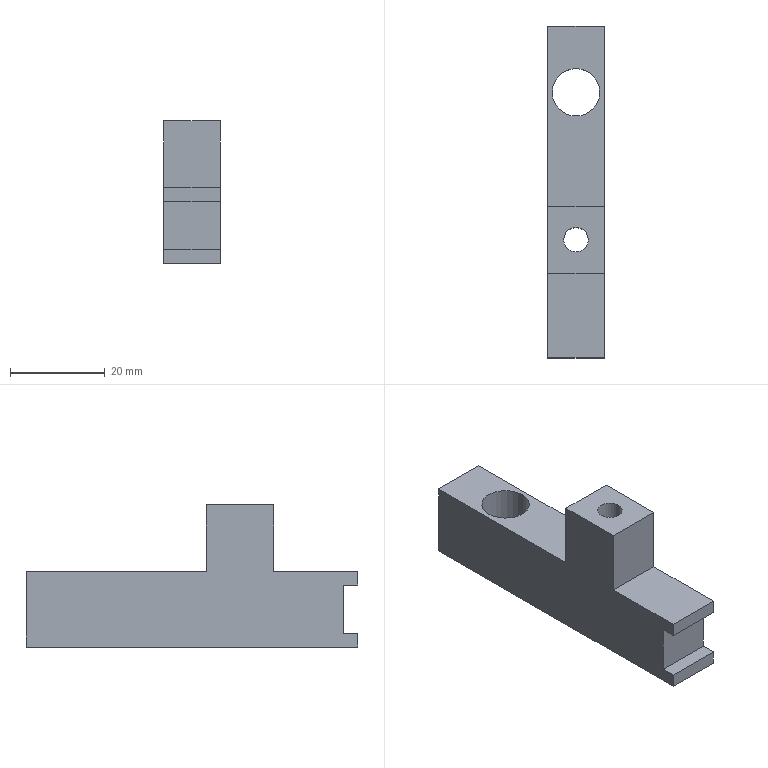Component | SolidWorks | JCT-03-03SwingBlock-1 | 1 solid | 18 faces | box 12 x 70 x 30 mm | volume 13565 mm3 | plane 14 | cylinder 4 | commonest cylinder face diameters 10 x2 5.2 x2
build123d program:
from build123d import *

# Parameters (mm, degrees)
EXTRUDE1_DEPTH     = 6
SKETCH2_R          = 2.6
EXTRUDE2_DEPTH     = 77.394
M10_TAPPED_HOLE1_D = 10


with BuildPart() as part:
    # Sketch1 → Extrude1 (new, symmetric)
    with BuildSketch(Plane(origin=(0, 0, 0), x_dir=(0, 0, -1), z_dir=(1, 0, 0))):
        Polygon((0, 0), (0, 70), (-16, 70), (-16, 32), (-30, 32), (-30, 17.8), (-16, 17.8), (-16, 0), (-13.1, 0), (-13.1, 3), (-2.9, 3), (-2.9, 0), align=None)
    extrude(amount=EXTRUDE1_DEPTH, both=True)

    # Sketch2 → Extrude2 (cut, through all)
    with BuildSketch(Plane.XY.offset(30)):
        with Locations((0, 24.9)):
            Circle(SKETCH2_R)
    extrude(amount=-EXTRUDE2_DEPTH, mode=Mode.SUBTRACT)

    # M10 Tapped Hole1 (through all)
    with Locations(Plane(origin=(0, 0, 0), x_dir=(-1, 0, 0), z_dir=(0, 0, -1))):
        with Locations((0, 56)):
            Hole(M10_TAPPED_HOLE1_D / 2)


solid = part.part

# Placed as in the assembly
solid = solid.moved(Location((7.266, 13.399, 26), (0, 0, 0)))
STEP:
#1=COLOUR_RGB('',0.7922,0.8196,0.9333);
#2=FILL_AREA_STYLE_COLOUR('',#1);
#3=FILL_AREA_STYLE('',(#2));
#4=SURFACE_STYLE_FILL_AREA(#3);
#5=SURFACE_SIDE_STYLE('',(#4));
#6=SURFACE_STYLE_USAGE(.BOTH.,#5);
#7=PRESENTATION_STYLE_ASSIGNMENT((#6));
#8=CARTESIAN_POINT('',(0.4829,2.732,1.654));
#9=VERTEX_POINT('',#8);
#10=CARTESIAN_POINT('',(0.08922,2.732,1.654));
#11=VERTEX_POINT('',#10);
#12=CARTESIAN_POINT('',(0.2861,2.732,1.654));
#13=DIRECTION('',(0.,0.,-1.));
#14=DIRECTION('',(-1.,0.,0.));
#15=AXIS2_PLACEMENT_3D('',#12,#13,#14);
#16=CIRCLE('',#15,0.1969);
#17=EDGE_CURVE('',#9,#11,#16,.T.);
#18=ORIENTED_EDGE('',*,*,#17,.F.);
#19=CARTESIAN_POINT('',(0.4829,2.732,1.024));
#20=VERTEX_POINT('',#19);
#21=CARTESIAN_POINT('',(0.4829,2.732,1.024));
#22=DIRECTION('',(0.,0.,-1.));
#23=VECTOR('',#22,39.37);
#24=LINE('',#21,#23);
#25=EDGE_CURVE('',#9,#20,#24,.T.);
#26=ORIENTED_EDGE('',*,*,#25,.T.);
#27=CARTESIAN_POINT('',(0.08922,2.732,1.024));
#28=VERTEX_POINT('',#27);
#29=CARTESIAN_POINT('',(0.2861,2.732,1.024));
#30=DIRECTION('',(0.,0.,-1.));
#31=DIRECTION('',(-1.,0.,0.));
#32=AXIS2_PLACEMENT_3D('',#29,#30,#31);
#33=CIRCLE('',#32,0.1969);
#34=EDGE_CURVE('',#20,#28,#33,.T.);
#35=ORIENTED_EDGE('',*,*,#34,.T.);
#36=CARTESIAN_POINT('',(0.08922,2.732,1.024));
#37=DIRECTION('',(0.,0.,-1.));
#38=VECTOR('',#37,39.37);
#39=LINE('',#36,#38);
#40=EDGE_CURVE('',#11,#28,#39,.T.);
#41=ORIENTED_EDGE('',*,*,#40,.F.);
#42=EDGE_LOOP('',(#18,#26,#35,#41));
#43=FACE_OUTER_BOUND('',#42,.T.);
#44=CARTESIAN_POINT('',(0.2861,2.732,1.024));
#45=DIRECTION('',(0.,0.,-1.));
#46=DIRECTION('',(-1.,0.,0.));
#47=AXIS2_PLACEMENT_3D('',#44,#45,#46);
#48=CYLINDRICAL_SURFACE('',#47,0.1969);
#49=ADVANCED_FACE('',(#43),#48,.F.);
#50=CARTESIAN_POINT('',(0.1837,1.508,1.024));
#51=VERTEX_POINT('',#50);
#52=CARTESIAN_POINT('',(0.3884,1.508,1.024));
#53=VERTEX_POINT('',#52);
#54=CARTESIAN_POINT('',(0.2861,1.508,1.024));
#55=DIRECTION('',(0.,0.,1.));
#56=DIRECTION('',(1.,0.,0.));
#57=AXIS2_PLACEMENT_3D('',#54,#55,#56);
#58=CIRCLE('',#57,0.1024);
#59=EDGE_CURVE('',#51,#53,#58,.T.);
#60=ORIENTED_EDGE('',*,*,#59,.F.);
#61=CARTESIAN_POINT('',(0.1837,1.508,2.205));
#62=VERTEX_POINT('',#61);
#63=CARTESIAN_POINT('',(0.1837,1.508,1.024));
#64=DIRECTION('',(0.,0.,1.));
#65=VECTOR('',#64,39.37);
#66=LINE('',#63,#65);
#67=EDGE_CURVE('',#51,#62,#66,.T.);
#68=ORIENTED_EDGE('',*,*,#67,.T.);
#69=CARTESIAN_POINT('',(0.3884,1.508,2.205));
#70=VERTEX_POINT('',#69);
#71=CARTESIAN_POINT('',(0.2861,1.508,2.205));
#72=DIRECTION('',(0.,0.,1.));
#73=DIRECTION('',(1.,0.,0.));
#74=AXIS2_PLACEMENT_3D('',#71,#72,#73);
#75=CIRCLE('',#74,0.1024);
#76=EDGE_CURVE('',#62,#70,#75,.T.);
#77=ORIENTED_EDGE('',*,*,#76,.T.);
#78=CARTESIAN_POINT('',(0.3884,1.508,1.024));
#79=DIRECTION('',(0.,0.,1.));
#80=VECTOR('',#79,39.37);
#81=LINE('',#78,#80);
#82=EDGE_CURVE('',#53,#70,#81,.T.);
#83=ORIENTED_EDGE('',*,*,#82,.F.);
#84=EDGE_LOOP('',(#60,#68,#77,#83));
#85=FACE_OUTER_BOUND('',#84,.T.);
#86=CARTESIAN_POINT('',(0.2861,1.508,1.024));
#87=DIRECTION('',(0.,0.,1.));
#88=DIRECTION('',(1.,0.,0.));
#89=AXIS2_PLACEMENT_3D('',#86,#87,#88);
#90=CYLINDRICAL_SURFACE('',#89,0.1024);
#91=ADVANCED_FACE('',(#85),#90,.F.);
#92=CARTESIAN_POINT('',(0.04985,0.5275,1.138));
#93=VERTEX_POINT('',#92);
#94=CARTESIAN_POINT('',(0.04985,0.5275,1.024));
#95=VERTEX_POINT('',#94);
#96=CARTESIAN_POINT('',(0.04985,0.5275,1.138));
#97=DIRECTION('',(0.,-0.,-1.));
#98=VECTOR('',#97,39.37);
#99=LINE('',#96,#98);
#100=EDGE_CURVE('',#93,#95,#99,.T.);
#101=ORIENTED_EDGE('',*,*,#100,.T.);
#102=CARTESIAN_POINT('',(0.5223,0.5275,1.024));
#103=VERTEX_POINT('',#102);
#104=CARTESIAN_POINT('',(0.5223,0.5275,1.024));
#105=DIRECTION('',(-1.,0.,0.));
#106=VECTOR('',#105,39.37);
#107=LINE('',#104,#106);
#108=EDGE_CURVE('',#103,#95,#107,.T.);
#109=ORIENTED_EDGE('',*,*,#108,.F.);
#110=CARTESIAN_POINT('',(0.5223,0.5275,1.138));
#111=VERTEX_POINT('',#110);
#112=CARTESIAN_POINT('',(0.5223,0.5275,1.138));
#113=DIRECTION('',(0.,-0.,-1.));
#114=VECTOR('',#113,39.37);
#115=LINE('',#112,#114);
#116=EDGE_CURVE('',#111,#103,#115,.T.);
#117=ORIENTED_EDGE('',*,*,#116,.F.);
#118=CARTESIAN_POINT('',(0.5223,0.5275,1.138));
#119=DIRECTION('',(-1.,0.,0.));
#120=VECTOR('',#119,39.37);
#121=LINE('',#118,#120);
#122=EDGE_CURVE('',#111,#93,#121,.T.);
#123=ORIENTED_EDGE('',*,*,#122,.T.);
#124=EDGE_LOOP('',(#101,#109,#117,#123));
#125=FACE_OUTER_BOUND('',#124,.T.);
#126=CARTESIAN_POINT('',(0.5223,0.5275,1.138));
#127=DIRECTION('',(0.,1.,-0.));
#128=DIRECTION('',(0.,0.,1.));
#129=AXIS2_PLACEMENT_3D('',#126,#127,#128);
#130=PLANE('',#129);
#131=ADVANCED_FACE('',(#125),#130,.F.);
#132=CARTESIAN_POINT('',(0.2861,2.732,1.024));
#133=DIRECTION('',(0.,0.,-1.));
#134=DIRECTION('',(-1.,0.,0.));
#135=AXIS2_PLACEMENT_3D('',#132,#133,#134);
#136=CIRCLE('',#135,0.1969);
#137=EDGE_CURVE('',#28,#20,#136,.T.);
#138=ORIENTED_EDGE('',*,*,#137,.F.);
#139=ORIENTED_EDGE('',*,*,#34,.F.);
#140=EDGE_LOOP('',(#138,#139));
#141=FACE_BOUND('',#140,.T.);
#142=CARTESIAN_POINT('',(0.2861,1.508,1.024));
#143=DIRECTION('',(0.,0.,1.));
#144=DIRECTION('',(1.,0.,0.));
#145=AXIS2_PLACEMENT_3D('',#142,#143,#144);
#146=CIRCLE('',#145,0.1024);
#147=EDGE_CURVE('',#53,#51,#146,.T.);
#148=ORIENTED_EDGE('',*,*,#147,.T.);
#149=ORIENTED_EDGE('',*,*,#59,.T.);
#150=EDGE_LOOP('',(#148,#149));
#151=FACE_BOUND('',#150,.T.);
#152=CARTESIAN_POINT('',(0.04985,3.283,1.024));
#153=VERTEX_POINT('',#152);
#154=CARTESIAN_POINT('',(0.04985,0.5275,1.024));
#155=DIRECTION('',(0.,1.,0.));
#156=VECTOR('',#155,39.37);
#157=LINE('',#154,#156);
#158=EDGE_CURVE('',#95,#153,#157,.T.);
#159=ORIENTED_EDGE('',*,*,#158,.T.);
#160=CARTESIAN_POINT('',(0.5223,3.283,1.024));
#161=VERTEX_POINT('',#160);
#162=CARTESIAN_POINT('',(0.5223,3.283,1.024));
#163=DIRECTION('',(-1.,0.,0.));
#164=VECTOR('',#163,39.37);
#165=LINE('',#162,#164);
#166=EDGE_CURVE('',#161,#153,#165,.T.);
#167=ORIENTED_EDGE('',*,*,#166,.F.);
#168=CARTESIAN_POINT('',(0.5223,0.5275,1.024));
#169=DIRECTION('',(0.,1.,0.));
#170=VECTOR('',#169,39.37);
#171=LINE('',#168,#170);
#172=EDGE_CURVE('',#103,#161,#171,.T.);
#173=ORIENTED_EDGE('',*,*,#172,.F.);
#174=ORIENTED_EDGE('',*,*,#108,.T.);
#175=EDGE_LOOP('',(#159,#167,#173,#174));
#176=FACE_OUTER_BOUND('',#175,.T.);
#177=CARTESIAN_POINT('',(0.5223,0.5275,1.024));
#178=DIRECTION('',(0.,0.,1.));
#179=DIRECTION('',(1.,0.,0.));
#180=AXIS2_PLACEMENT_3D('',#177,#178,#179);
#181=PLANE('',#180);
#182=ADVANCED_FACE('',(#141,#151,#176),#181,.F.);
#183=CARTESIAN_POINT('',(0.04985,3.283,1.654));
#184=VERTEX_POINT('',#183);
#185=CARTESIAN_POINT('',(0.04985,3.283,1.024));
#186=DIRECTION('',(0.,0.,1.));
#187=VECTOR('',#186,39.37);
#188=LINE('',#185,#187);
#189=EDGE_CURVE('',#153,#184,#188,.T.);
#190=ORIENTED_EDGE('',*,*,#189,.T.);
#191=CARTESIAN_POINT('',(0.5223,3.283,1.654));
#192=VERTEX_POINT('',#191);
#193=CARTESIAN_POINT('',(0.5223,3.283,1.654));
#194=DIRECTION('',(-1.,0.,0.));
#195=VECTOR('',#194,39.37);
#196=LINE('',#193,#195);
#197=EDGE_CURVE('',#192,#184,#196,.T.);
#198=ORIENTED_EDGE('',*,*,#197,.F.);
#199=CARTESIAN_POINT('',(0.5223,3.283,1.024));
#200=DIRECTION('',(0.,0.,1.));
#201=VECTOR('',#200,39.37);
#202=LINE('',#199,#201);
#203=EDGE_CURVE('',#161,#192,#202,.T.);
#204=ORIENTED_EDGE('',*,*,#203,.F.);
#205=ORIENTED_EDGE('',*,*,#166,.T.);
#206=EDGE_LOOP('',(#190,#198,#204,#205));
#207=FACE_OUTER_BOUND('',#206,.T.);
#208=CARTESIAN_POINT('',(0.5223,3.283,1.024));
#209=DIRECTION('',(0.,-1.,0.));
#210=DIRECTION('',(0.,0.,-1.));
#211=AXIS2_PLACEMENT_3D('',#208,#209,#210);
#212=PLANE('',#211);
#213=ADVANCED_FACE('',(#207),#212,.F.);
#214=CARTESIAN_POINT('',(0.2861,2.732,1.654));
#215=DIRECTION('',(0.,0.,-1.));
#216=DIRECTION('',(-1.,0.,0.));
#217=AXIS2_PLACEMENT_3D('',#214,#215,#216);
#218=CIRCLE('',#217,0.1969);
#219=EDGE_CURVE('',#11,#9,#218,.T.);
#220=ORIENTED_EDGE('',*,*,#219,.T.);
#221=ORIENTED_EDGE('',*,*,#17,.T.);
#222=EDGE_LOOP('',(#220,#221));
#223=FACE_BOUND('',#222,.T.);
#224=CARTESIAN_POINT('',(0.04985,1.787,1.654));
#225=VERTEX_POINT('',#224);
#226=CARTESIAN_POINT('',(0.04985,3.283,1.654));
#227=DIRECTION('',(0.,-1.,0.));
#228=VECTOR('',#227,39.37);
#229=LINE('',#226,#228);
#230=EDGE_CURVE('',#184,#225,#229,.T.);
#231=ORIENTED_EDGE('',*,*,#230,.T.);
#232=CARTESIAN_POINT('',(0.5223,1.787,1.654));
#233=VERTEX_POINT('',#232);
#234=CARTESIAN_POINT('',(0.5223,1.787,1.654));
#235=DIRECTION('',(-1.,0.,0.));
#236=VECTOR('',#235,39.37);
#237=LINE('',#234,#236);
#238=EDGE_CURVE('',#233,#225,#237,.T.);
#239=ORIENTED_EDGE('',*,*,#238,.F.);
#240=CARTESIAN_POINT('',(0.5223,3.283,1.654));
#241=DIRECTION('',(0.,-1.,0.));
#242=VECTOR('',#241,39.37);
#243=LINE('',#240,#242);
#244=EDGE_CURVE('',#192,#233,#243,.T.);
#245=ORIENTED_EDGE('',*,*,#244,.F.);
#246=ORIENTED_EDGE('',*,*,#197,.T.);
#247=EDGE_LOOP('',(#231,#239,#245,#246));
#248=FACE_OUTER_BOUND('',#247,.T.);
#249=CARTESIAN_POINT('',(0.5223,3.283,1.654));
#250=DIRECTION('',(0.,0.,-1.));
#251=DIRECTION('',(-1.,0.,0.));
#252=AXIS2_PLACEMENT_3D('',#249,#250,#251);
#253=PLANE('',#252);
#254=ADVANCED_FACE('',(#223,#248),#253,.F.);
#255=CARTESIAN_POINT('',(0.04985,1.787,2.205));
#256=VERTEX_POINT('',#255);
#257=CARTESIAN_POINT('',(0.04985,1.787,1.654));
#258=DIRECTION('',(0.,0.,1.));
#259=VECTOR('',#258,39.37);
#260=LINE('',#257,#259);
#261=EDGE_CURVE('',#225,#256,#260,.T.);
#262=ORIENTED_EDGE('',*,*,#261,.T.);
#263=CARTESIAN_POINT('',(0.5223,1.787,2.205));
#264=VERTEX_POINT('',#263);
#265=CARTESIAN_POINT('',(0.5223,1.787,2.205));
#266=DIRECTION('',(-1.,0.,0.));
#267=VECTOR('',#266,39.37);
#268=LINE('',#265,#267);
#269=EDGE_CURVE('',#264,#256,#268,.T.);
#270=ORIENTED_EDGE('',*,*,#269,.F.);
#271=CARTESIAN_POINT('',(0.5223,1.787,1.654));
#272=DIRECTION('',(0.,0.,1.));
#273=VECTOR('',#272,39.37);
#274=LINE('',#271,#273);
#275=EDGE_CURVE('',#233,#264,#274,.T.);
#276=ORIENTED_EDGE('',*,*,#275,.F.);
#277=ORIENTED_EDGE('',*,*,#238,.T.);
#278=EDGE_LOOP('',(#262,#270,#276,#277));
#279=FACE_OUTER_BOUND('',#278,.T.);
#280=CARTESIAN_POINT('',(0.5223,1.787,1.654));
#281=DIRECTION('',(0.,-1.,0.));
#282=DIRECTION('',(0.,0.,-1.));
#283=AXIS2_PLACEMENT_3D('',#280,#281,#282);
#284=PLANE('',#283);
#285=ADVANCED_FACE('',(#279),#284,.F.);
#286=CARTESIAN_POINT('',(0.2861,1.508,2.205));
#287=DIRECTION('',(0.,0.,1.));
#288=DIRECTION('',(1.,0.,0.));
#289=AXIS2_PLACEMENT_3D('',#286,#287,#288);
#290=CIRCLE('',#289,0.1024);
#291=EDGE_CURVE('',#70,#62,#290,.T.);
#292=ORIENTED_EDGE('',*,*,#291,.F.);
#293=ORIENTED_EDGE('',*,*,#76,.F.);
#294=EDGE_LOOP('',(#292,#293));
#295=FACE_BOUND('',#294,.T.);
#296=CARTESIAN_POINT('',(0.04985,1.228,2.205));
#297=VERTEX_POINT('',#296);
#298=CARTESIAN_POINT('',(0.04985,1.787,2.205));
#299=DIRECTION('',(0.,-1.,0.));
#300=VECTOR('',#299,39.37);
#301=LINE('',#298,#300);
#302=EDGE_CURVE('',#256,#297,#301,.T.);
#303=ORIENTED_EDGE('',*,*,#302,.T.);
#304=CARTESIAN_POINT('',(0.5223,1.228,2.205));
#305=VERTEX_POINT('',#304);
#306=CARTESIAN_POINT('',(0.5223,1.228,2.205));
#307=DIRECTION('',(-1.,0.,0.));
#308=VECTOR('',#307,39.37);
#309=LINE('',#306,#308);
#310=EDGE_CURVE('',#305,#297,#309,.T.);
#311=ORIENTED_EDGE('',*,*,#310,.F.);
#312=CARTESIAN_POINT('',(0.5223,1.787,2.205));
#313=DIRECTION('',(0.,-1.,0.));
#314=VECTOR('',#313,39.37);
#315=LINE('',#312,#314);
#316=EDGE_CURVE('',#264,#305,#315,.T.);
#317=ORIENTED_EDGE('',*,*,#316,.F.);
#318=ORIENTED_EDGE('',*,*,#269,.T.);
#319=EDGE_LOOP('',(#303,#311,#317,#318));
#320=FACE_OUTER_BOUND('',#319,.T.);
#321=CARTESIAN_POINT('',(0.5223,1.787,2.205));
#322=DIRECTION('',(0.,0.,-1.));
#323=DIRECTION('',(-1.,0.,0.));
#324=AXIS2_PLACEMENT_3D('',#321,#322,#323);
#325=PLANE('',#324);
#326=ADVANCED_FACE('',(#295,#320),#325,.F.);
#327=CARTESIAN_POINT('',(0.04985,1.228,1.654));
#328=VERTEX_POINT('',#327);
#329=CARTESIAN_POINT('',(0.04985,1.228,2.205));
#330=DIRECTION('',(0.,0.,-1.));
#331=VECTOR('',#330,39.37);
#332=LINE('',#329,#331);
#333=EDGE_CURVE('',#297,#328,#332,.T.);
#334=ORIENTED_EDGE('',*,*,#333,.T.);
#335=CARTESIAN_POINT('',(0.5223,1.228,1.654));
#336=VERTEX_POINT('',#335);
#337=CARTESIAN_POINT('',(0.5223,1.228,1.654));
#338=DIRECTION('',(-1.,0.,0.));
#339=VECTOR('',#338,39.37);
#340=LINE('',#337,#339);
#341=EDGE_CURVE('',#336,#328,#340,.T.);
#342=ORIENTED_EDGE('',*,*,#341,.F.);
#343=CARTESIAN_POINT('',(0.5223,1.228,2.205));
#344=DIRECTION('',(0.,0.,-1.));
#345=VECTOR('',#344,39.37);
#346=LINE('',#343,#345);
#347=EDGE_CURVE('',#305,#336,#346,.T.);
#348=ORIENTED_EDGE('',*,*,#347,.F.);
#349=ORIENTED_EDGE('',*,*,#310,.T.);
#350=EDGE_LOOP('',(#334,#342,#348,#349));
#351=FACE_OUTER_BOUND('',#350,.T.);
#352=CARTESIAN_POINT('',(0.5223,1.228,2.205));
#353=DIRECTION('',(0.,1.,0.));
#354=DIRECTION('',(0.,0.,1.));
#355=AXIS2_PLACEMENT_3D('',#352,#353,#354);
#356=PLANE('',#355);
#357=ADVANCED_FACE('',(#351),#356,.F.);
#358=CARTESIAN_POINT('',(0.04985,0.5275,1.654));
#359=VERTEX_POINT('',#358);
#360=CARTESIAN_POINT('',(0.04985,1.228,1.654));
#361=DIRECTION('',(0.,-1.,-0.));
#362=VECTOR('',#361,39.37);
#363=LINE('',#360,#362);
#364=EDGE_CURVE('',#328,#359,#363,.T.);
#365=ORIENTED_EDGE('',*,*,#364,.T.);
#366=CARTESIAN_POINT('',(0.5223,0.5275,1.654));
#367=VERTEX_POINT('',#366);
#368=CARTESIAN_POINT('',(0.5223,0.5275,1.654));
#369=DIRECTION('',(-1.,0.,0.));
#370=VECTOR('',#369,39.37);
#371=LINE('',#368,#370);
#372=EDGE_CURVE('',#367,#359,#371,.T.);
#373=ORIENTED_EDGE('',*,*,#372,.F.);
#374=CARTESIAN_POINT('',(0.5223,1.228,1.654));
#375=DIRECTION('',(0.,-1.,-0.));
#376=VECTOR('',#375,39.37);
#377=LINE('',#374,#376);
#378=EDGE_CURVE('',#336,#367,#377,.T.);
#379=ORIENTED_EDGE('',*,*,#378,.F.);
#380=ORIENTED_EDGE('',*,*,#341,.T.);
#381=EDGE_LOOP('',(#365,#373,#379,#380));
#382=FACE_OUTER_BOUND('',#381,.T.);
#383=CARTESIAN_POINT('',(0.5223,1.228,1.654));
#384=DIRECTION('',(0.,0.,-1.));
#385=DIRECTION('',(0.,1.,0.));
#386=AXIS2_PLACEMENT_3D('',#383,#384,#385);
#387=PLANE('',#386);
#388=ADVANCED_FACE('',(#382),#387,.F.);
#389=CARTESIAN_POINT('',(0.04985,0.5275,1.539));
#390=VERTEX_POINT('',#389);
#391=CARTESIAN_POINT('',(0.04985,0.5275,1.654));
#392=DIRECTION('',(0.,0.,-1.));
#393=VECTOR('',#392,39.37);
#394=LINE('',#391,#393);
#395=EDGE_CURVE('',#359,#390,#394,.T.);
#396=ORIENTED_EDGE('',*,*,#395,.T.);
#397=CARTESIAN_POINT('',(0.5223,0.5275,1.539));
#398=VERTEX_POINT('',#397);
#399=CARTESIAN_POINT('',(0.5223,0.5275,1.539));
#400=DIRECTION('',(-1.,0.,0.));
#401=VECTOR('',#400,39.37);
#402=LINE('',#399,#401);
#403=EDGE_CURVE('',#398,#390,#402,.T.);
#404=ORIENTED_EDGE('',*,*,#403,.F.);
#405=CARTESIAN_POINT('',(0.5223,0.5275,1.654));
#406=DIRECTION('',(0.,0.,-1.));
#407=VECTOR('',#406,39.37);
#408=LINE('',#405,#407);
#409=EDGE_CURVE('',#367,#398,#408,.T.);
#410=ORIENTED_EDGE('',*,*,#409,.F.);
#411=ORIENTED_EDGE('',*,*,#372,.T.);
#412=EDGE_LOOP('',(#396,#404,#410,#411));
#413=FACE_OUTER_BOUND('',#412,.T.);
#414=CARTESIAN_POINT('',(0.5223,0.5275,1.654));
#415=DIRECTION('',(0.,1.,0.));
#416=DIRECTION('',(0.,0.,1.));
#417=AXIS2_PLACEMENT_3D('',#414,#415,#416);
#418=PLANE('',#417);
#419=ADVANCED_FACE('',(#413),#418,.F.);
#420=CARTESIAN_POINT('',(0.04985,0.6456,1.539));
#421=VERTEX_POINT('',#420);
#422=CARTESIAN_POINT('',(0.04985,0.5275,1.539));
#423=DIRECTION('',(0.,1.,0.));
#424=VECTOR('',#423,39.37);
#425=LINE('',#422,#424);
#426=EDGE_CURVE('',#390,#421,#425,.T.);
#427=ORIENTED_EDGE('',*,*,#426,.T.);
#428=CARTESIAN_POINT('',(0.5223,0.6456,1.539));
#429=VERTEX_POINT('',#428);
#430=CARTESIAN_POINT('',(0.5223,0.6456,1.539));
#431=DIRECTION('',(-1.,0.,0.));
#432=VECTOR('',#431,39.37);
#433=LINE('',#430,#432);
#434=EDGE_CURVE('',#429,#421,#433,.T.);
#435=ORIENTED_EDGE('',*,*,#434,.F.);
#436=CARTESIAN_POINT('',(0.5223,0.5275,1.539));
#437=DIRECTION('',(0.,1.,0.));
#438=VECTOR('',#437,39.37);
#439=LINE('',#436,#438);
#440=EDGE_CURVE('',#398,#429,#439,.T.);
#441=ORIENTED_EDGE('',*,*,#440,.F.);
#442=ORIENTED_EDGE('',*,*,#403,.T.);
#443=EDGE_LOOP('',(#427,#435,#441,#442));
#444=FACE_OUTER_BOUND('',#443,.T.);
#445=CARTESIAN_POINT('',(0.5223,0.5275,1.539));
#446=DIRECTION('',(0.,0.,1.));
#447=DIRECTION('',(1.,0.,0.));
#448=AXIS2_PLACEMENT_3D('',#445,#446,#447);
#449=PLANE('',#448);
#450=ADVANCED_FACE('',(#444),#449,.F.);
#451=CARTESIAN_POINT('',(0.04985,0.6456,1.138));
#452=VERTEX_POINT('',#451);
#453=CARTESIAN_POINT('',(0.04985,0.6456,1.539));
#454=DIRECTION('',(0.,0.,-1.));
#455=VECTOR('',#454,39.37);
#456=LINE('',#453,#455);
#457=EDGE_CURVE('',#421,#452,#456,.T.);
#458=ORIENTED_EDGE('',*,*,#457,.T.);
#459=CARTESIAN_POINT('',(0.5223,0.6456,1.138));
#460=VERTEX_POINT('',#459);
#461=CARTESIAN_POINT('',(0.5223,0.6456,1.138));
#462=DIRECTION('',(-1.,0.,0.));
#463=VECTOR('',#462,39.37);
#464=LINE('',#461,#463);
#465=EDGE_CURVE('',#460,#452,#464,.T.);
#466=ORIENTED_EDGE('',*,*,#465,.F.);
#467=CARTESIAN_POINT('',(0.5223,0.6456,1.539));
#468=DIRECTION('',(0.,0.,-1.));
#469=VECTOR('',#468,39.37);
#470=LINE('',#467,#469);
#471=EDGE_CURVE('',#429,#460,#470,.T.);
#472=ORIENTED_EDGE('',*,*,#471,.F.);
#473=ORIENTED_EDGE('',*,*,#434,.T.);
#474=EDGE_LOOP('',(#458,#466,#472,#473));
#475=FACE_OUTER_BOUND('',#474,.T.);
#476=CARTESIAN_POINT('',(0.5223,0.6456,1.539));
#477=DIRECTION('',(0.,1.,0.));
#478=DIRECTION('',(0.,-0.,1.));
#479=AXIS2_PLACEMENT_3D('',#476,#477,#478);
#480=PLANE('',#479);
#481=ADVANCED_FACE('',(#475),#480,.F.);
#482=CARTESIAN_POINT('',(0.04985,0.6456,1.138));
#483=DIRECTION('',(0.,-1.,-0.));
#484=VECTOR('',#483,39.37);
#485=LINE('',#482,#484);
#486=EDGE_CURVE('',#452,#93,#485,.T.);
#487=ORIENTED_EDGE('',*,*,#486,.T.);
#488=ORIENTED_EDGE('',*,*,#122,.F.);
#489=CARTESIAN_POINT('',(0.5223,0.6456,1.138));
#490=DIRECTION('',(0.,-1.,-0.));
#491=VECTOR('',#490,39.37);
#492=LINE('',#489,#491);
#493=EDGE_CURVE('',#460,#111,#492,.T.);
#494=ORIENTED_EDGE('',*,*,#493,.F.);
#495=ORIENTED_EDGE('',*,*,#465,.T.);
#496=EDGE_LOOP('',(#487,#488,#494,#495));
#497=FACE_OUTER_BOUND('',#496,.T.);
#498=CARTESIAN_POINT('',(0.5223,0.6456,1.138));
#499=DIRECTION('',(0.,0.,-1.));
#500=DIRECTION('',(0.,1.,0.));
#501=AXIS2_PLACEMENT_3D('',#498,#499,#500);
#502=PLANE('',#501);
#503=ADVANCED_FACE('',(#497),#502,.F.);
#504=ORIENTED_EDGE('',*,*,#116,.T.);
#505=ORIENTED_EDGE('',*,*,#172,.T.);
#506=ORIENTED_EDGE('',*,*,#203,.T.);
#507=ORIENTED_EDGE('',*,*,#244,.T.);
#508=ORIENTED_EDGE('',*,*,#275,.T.);
#509=ORIENTED_EDGE('',*,*,#316,.T.);
#510=ORIENTED_EDGE('',*,*,#347,.T.);
#511=ORIENTED_EDGE('',*,*,#378,.T.);
#512=ORIENTED_EDGE('',*,*,#409,.T.);
#513=ORIENTED_EDGE('',*,*,#440,.T.);
#514=ORIENTED_EDGE('',*,*,#471,.T.);
#515=ORIENTED_EDGE('',*,*,#493,.T.);
#516=EDGE_LOOP('',(#504,#505,#506,#507,#508,#509,#510,#511,#512,#513,#514,#515));
#517=FACE_OUTER_BOUND('',#516,.T.);
#518=CARTESIAN_POINT('',(0.5223,0.5275,1.024));
#519=DIRECTION('',(1.,0.,0.));
#520=DIRECTION('',(0.,0.,-1.));
#521=AXIS2_PLACEMENT_3D('',#518,#519,#520);
#522=PLANE('',#521);
#523=ADVANCED_FACE('',(#517),#522,.T.);
#524=ORIENTED_EDGE('',*,*,#100,.F.);
#525=ORIENTED_EDGE('',*,*,#486,.F.);
#526=ORIENTED_EDGE('',*,*,#457,.F.);
#527=ORIENTED_EDGE('',*,*,#426,.F.);
#528=ORIENTED_EDGE('',*,*,#395,.F.);
#529=ORIENTED_EDGE('',*,*,#364,.F.);
#530=ORIENTED_EDGE('',*,*,#333,.F.);
#531=ORIENTED_EDGE('',*,*,#302,.F.);
#532=ORIENTED_EDGE('',*,*,#261,.F.);
#533=ORIENTED_EDGE('',*,*,#230,.F.);
#534=ORIENTED_EDGE('',*,*,#189,.F.);
#535=ORIENTED_EDGE('',*,*,#158,.F.);
#536=EDGE_LOOP('',(#524,#525,#526,#527,#528,#529,#530,#531,#532,#533,#534,#535));
#537=FACE_OUTER_BOUND('',#536,.T.);
#538=CARTESIAN_POINT('',(0.04985,0.5275,1.024));
#539=DIRECTION('',(1.,0.,0.));
#540=DIRECTION('',(0.,0.,-1.));
#541=AXIS2_PLACEMENT_3D('',#538,#539,#540);
#542=PLANE('',#541);
#543=ADVANCED_FACE('',(#537),#542,.F.);
#544=ORIENTED_EDGE('',*,*,#67,.F.);
#545=ORIENTED_EDGE('',*,*,#147,.F.);
#546=ORIENTED_EDGE('',*,*,#82,.T.);
#547=ORIENTED_EDGE('',*,*,#291,.T.);
#548=EDGE_LOOP('',(#544,#545,#546,#547));
#549=FACE_OUTER_BOUND('',#548,.T.);
#550=CARTESIAN_POINT('',(0.2861,1.508,1.024));
#551=DIRECTION('',(0.,0.,1.));
#552=DIRECTION('',(1.,0.,0.));
#553=AXIS2_PLACEMENT_3D('',#550,#551,#552);
#554=CYLINDRICAL_SURFACE('',#553,0.1024);
#555=ADVANCED_FACE('',(#549),#554,.F.);
#556=ORIENTED_EDGE('',*,*,#25,.F.);
#557=ORIENTED_EDGE('',*,*,#219,.F.);
#558=ORIENTED_EDGE('',*,*,#40,.T.);
#559=ORIENTED_EDGE('',*,*,#137,.T.);
#560=EDGE_LOOP('',(#556,#557,#558,#559));
#561=FACE_OUTER_BOUND('',#560,.T.);
#562=CARTESIAN_POINT('',(0.2861,2.732,1.024));
#563=DIRECTION('',(0.,0.,-1.));
#564=DIRECTION('',(-1.,0.,0.));
#565=AXIS2_PLACEMENT_3D('',#562,#563,#564);
#566=CYLINDRICAL_SURFACE('',#565,0.1969);
#567=ADVANCED_FACE('',(#561),#566,.F.);
#568=CLOSED_SHELL('',(#49,#91,#131,#182,#213,#254,#285,#326,#357,#388,#419,#450,#481,#503,#523,#543,#555,#567));
#569=MANIFOLD_SOLID_BREP('',#568);
#570=STYLED_ITEM('',(#7),#569);
#571=PRESENTATION_LAYER_ASSIGNMENT('','',(#570));
#572=(LENGTH_UNIT()NAMED_UNIT(*)SI_UNIT($,.METRE.));
#573=LENGTH_MEASURE_WITH_UNIT(LENGTH_MEASURE(0.0254),#572);
#574=DIMENSIONAL_EXPONENTS(1.,0.,0.,0.,0.,0.,0.);
#575=(CONVERSION_BASED_UNIT('',#573)LENGTH_UNIT()NAMED_UNIT(#574));
#576=UNCERTAINTY_MEASURE_WITH_UNIT(LENGTH_MEASURE(0.00001),#575,'','');
#577=(NAMED_UNIT(*)PLANE_ANGLE_UNIT()SI_UNIT($,.RADIAN.));
#578=(NAMED_UNIT(*)SI_UNIT($,.STERADIAN.)SOLID_ANGLE_UNIT());
#579=(GEOMETRIC_REPRESENTATION_CONTEXT(3)GLOBAL_UNCERTAINTY_ASSIGNED_CONTEXT((#576))GLOBAL_UNIT_ASSIGNED_CONTEXT((#575,#577,#578))REPRESENTATION_CONTEXT('',''));
#580=MECHANICAL_DESIGN_GEOMETRIC_PRESENTATION_REPRESENTATION('',(#570),#579);
#581=CARTESIAN_POINT('',(0.,0.,0.));
#582=DIRECTION('',(0.,0.,1.));
#583=DIRECTION('',(1.,0.,0.));
#584=AXIS2_PLACEMENT_3D('',#581,#582,#583);
#585=(LENGTH_UNIT()NAMED_UNIT(*)SI_UNIT($,.METRE.));
#586=LENGTH_MEASURE_WITH_UNIT(LENGTH_MEASURE(0.0254),#585);
#587=DIMENSIONAL_EXPONENTS(1.,0.,0.,0.,0.,0.,0.);
#588=(CONVERSION_BASED_UNIT('',#586)LENGTH_UNIT()NAMED_UNIT(#587));
#589=UNCERTAINTY_MEASURE_WITH_UNIT(LENGTH_MEASURE(0.00001),#588,'','');
#590=(NAMED_UNIT(*)PLANE_ANGLE_UNIT()SI_UNIT($,.RADIAN.));
#591=(NAMED_UNIT(*)SI_UNIT($,.STERADIAN.)SOLID_ANGLE_UNIT());
#592=(GEOMETRIC_REPRESENTATION_CONTEXT(3)GLOBAL_UNCERTAINTY_ASSIGNED_CONTEXT((#589))GLOBAL_UNIT_ASSIGNED_CONTEXT((#588,#590,#591))REPRESENTATION_CONTEXT('',''));
#593=ADVANCED_BREP_SHAPE_REPRESENTATION('',(#569,#584),#592);